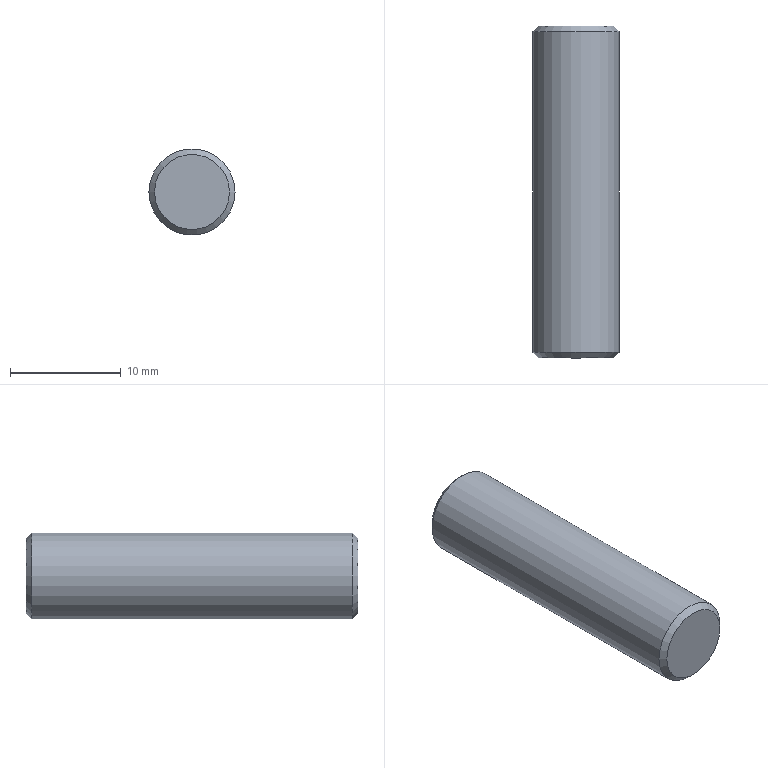Component | NX | STUD_2 | 1 solid | 5 faces | box 7.79 x 30 x 7.79 mm | volume 1422 mm3 | plane 2 | cone 2 | cylinder 1 | commonest cylinder face diameters 7.785 x1
STEP:
#1=CARTESIAN_POINT('',(0.,0.,0.));
#2=DIRECTION('',(0.,0.,1.));
#3=DIRECTION('',(1.,0.,0.));
#4=AXIS2_PLACEMENT_3D('',#1,#2,#3);
#5=CARTESIAN_POINT('',(-23.607,51.5,10.75));
#6=VERTEX_POINT('',#5);
#7=CARTESIAN_POINT('',(-27.,51.5,10.75));
#8=DIRECTION('',(0.,1.,0.));
#9=DIRECTION('',(1.,0.,0.));
#10=AXIS2_PLACEMENT_3D('',#7,#8,#9);
#11=CIRCLE('',#10,3.393);
#12=CARTESIAN_POINT('',(-27.,51.5,10.75));
#13=DIRECTION('',(0.,1.,0.));
#14=DIRECTION('',(1.,0.,0.));
#15=AXIS2_PLACEMENT_3D('',#12,#13,#14);
#16=PLANE('',#15);
#17=CARTESIAN_POINT('',(0.,0.));
#18=DIRECTION('',(1.,0.));
#19=AXIS2_PLACEMENT_2D('',#17,#18);
#20=CIRCLE('',#19,3.393);
#21=(GEOMETRIC_REPRESENTATION_CONTEXT(2)PARAMETRIC_REPRESENTATION_CONTEXT()REPRESENTATION_CONTEXT('',''));
#22=DEFINITIONAL_REPRESENTATION('',(#20),#21);
#23=PCURVE('',#16,#22);
#24=CARTESIAN_POINT('',(-27.,51.,10.75));
#25=DIRECTION('',(0.,-1.,0.));
#26=DIRECTION('',(-1.,0.,0.));
#27=AXIS2_PLACEMENT_3D('',#24,#25,#26);
#28=CONICAL_SURFACE('',#27,3.893,0.7854);
#29=CARTESIAN_POINT('',(9.425,-0.5));
#30=DIRECTION('',(-1.,0.));
#31=VECTOR('',#30,1.);
#32=LINE('',#29,#31);
#33=(GEOMETRIC_REPRESENTATION_CONTEXT(2)PARAMETRIC_REPRESENTATION_CONTEXT()REPRESENTATION_CONTEXT('',''));
#34=DEFINITIONAL_REPRESENTATION('',(#32),#33);
#35=PCURVE('',#28,#34);
#36=SURFACE_CURVE('',#11,(#23,#35),.PCURVE_S1.);
#37=EDGE_CURVE('',#6,#6,#36,.T.);
#38=ORIENTED_EDGE('',*,*,#37,.T.);
#39=EDGE_LOOP('',(#38));
#40=FACE_BOUND('',#39,.T.);
#41=ADVANCED_FACE('',(#40),#16,.T.);
#42=CARTESIAN_POINT('',(-30.393,21.5,10.75));
#43=VERTEX_POINT('',#42);
#44=CARTESIAN_POINT('',(-27.,21.5,10.75));
#45=DIRECTION('',(0.,-1.,0.));
#46=DIRECTION('',(-1.,0.,0.));
#47=AXIS2_PLACEMENT_3D('',#44,#45,#46);
#48=CIRCLE('',#47,3.393);
#49=CARTESIAN_POINT('',(-27.,21.5,10.75));
#50=DIRECTION('',(0.,-1.,0.));
#51=DIRECTION('',(-1.,0.,0.));
#52=AXIS2_PLACEMENT_3D('',#49,#50,#51);
#53=PLANE('',#52);
#54=CARTESIAN_POINT('',(0.,0.));
#55=DIRECTION('',(1.,0.));
#56=AXIS2_PLACEMENT_2D('',#54,#55);
#57=CIRCLE('',#56,3.393);
#58=(GEOMETRIC_REPRESENTATION_CONTEXT(2)PARAMETRIC_REPRESENTATION_CONTEXT()REPRESENTATION_CONTEXT('',''));
#59=DEFINITIONAL_REPRESENTATION('',(#57),#58);
#60=PCURVE('',#53,#59);
#61=CARTESIAN_POINT('',(-27.,22.,10.75));
#62=DIRECTION('',(0.,1.,0.));
#63=DIRECTION('',(1.,0.,0.));
#64=AXIS2_PLACEMENT_3D('',#61,#62,#63);
#65=CONICAL_SURFACE('',#64,3.893,0.7854);
#66=CARTESIAN_POINT('',(9.425,-0.5));
#67=DIRECTION('',(-1.,0.));
#68=VECTOR('',#67,1.);
#69=LINE('',#66,#68);
#70=(GEOMETRIC_REPRESENTATION_CONTEXT(2)PARAMETRIC_REPRESENTATION_CONTEXT()REPRESENTATION_CONTEXT('',''));
#71=DEFINITIONAL_REPRESENTATION('',(#69),#70);
#72=PCURVE('',#65,#71);
#73=SURFACE_CURVE('',#48,(#60,#72),.PCURVE_S1.);
#74=EDGE_CURVE('',#43,#43,#73,.T.);
#75=ORIENTED_EDGE('',*,*,#74,.T.);
#76=EDGE_LOOP('',(#75));
#77=FACE_BOUND('',#76,.T.);
#78=ADVANCED_FACE('',(#77),#53,.T.);
#79=CARTESIAN_POINT('',(-30.893,22.,10.75));
#80=VERTEX_POINT('',#79);
#81=CARTESIAN_POINT('',(-23.107,22.,10.75));
#82=VERTEX_POINT('',#81);
#83=CARTESIAN_POINT('',(-27.,22.,10.75));
#84=DIRECTION('',(0.,1.,0.));
#85=DIRECTION('',(-1.,0.,0.));
#86=AXIS2_PLACEMENT_3D('',#83,#84,#85);
#87=CIRCLE('',#86,3.893);
#88=CARTESIAN_POINT('',(-27.,21.5,10.75));
#89=DIRECTION('',(0.,1.,0.));
#90=DIRECTION('',(1.,0.,0.));
#91=AXIS2_PLACEMENT_3D('',#88,#89,#90);
#92=CYLINDRICAL_SURFACE('',#91,3.893);
#93=CARTESIAN_POINT('',(3.142,0.5));
#94=DIRECTION('',(1.,0.));
#95=VECTOR('',#94,1.);
#96=LINE('',#93,#95);
#97=(GEOMETRIC_REPRESENTATION_CONTEXT(2)PARAMETRIC_REPRESENTATION_CONTEXT()REPRESENTATION_CONTEXT('',''));
#98=DEFINITIONAL_REPRESENTATION('',(#96),#97);
#99=PCURVE('',#92,#98);
#100=CARTESIAN_POINT('',(3.142,0.));
#101=DIRECTION('',(1.,0.));
#102=VECTOR('',#101,1.);
#103=LINE('',#100,#102);
#104=(GEOMETRIC_REPRESENTATION_CONTEXT(2)PARAMETRIC_REPRESENTATION_CONTEXT()REPRESENTATION_CONTEXT('',''));
#105=DEFINITIONAL_REPRESENTATION('',(#103),#104);
#106=PCURVE('',#65,#105);
#107=SURFACE_CURVE('',#87,(#99,#106),.PCURVE_S1.);
#108=EDGE_CURVE('',#80,#82,#107,.T.);
#109=ORIENTED_EDGE('',*,*,#108,.T.);
#110=CARTESIAN_POINT('',(-23.107,51.,10.75));
#111=VERTEX_POINT('',#110);
#112=CARTESIAN_POINT('',(-23.107,22.,10.75));
#113=CARTESIAN_POINT('',(-23.107,51.,10.75));
#114=B_SPLINE_CURVE_WITH_KNOTS('',1,(#112,#113),.UNSPECIFIED.,.F.,.F.,(2,2),(0.5,29.5),.PIECEWISE_BEZIER_KNOTS.);
#115=CARTESIAN_POINT('',(6.283,0.));
#116=DIRECTION('',(0.,1.));
#117=VECTOR('',#116,1.);
#118=LINE('',#115,#117);
#119=(GEOMETRIC_REPRESENTATION_CONTEXT(2)PARAMETRIC_REPRESENTATION_CONTEXT()REPRESENTATION_CONTEXT('',''));
#120=DEFINITIONAL_REPRESENTATION('',(#118),#119);
#121=PCURVE('',#92,#120);
#122=CARTESIAN_POINT('',(0.,0.));
#123=DIRECTION('',(0.,1.));
#124=VECTOR('',#123,1.);
#125=LINE('',#122,#124);
#126=(GEOMETRIC_REPRESENTATION_CONTEXT(2)PARAMETRIC_REPRESENTATION_CONTEXT()REPRESENTATION_CONTEXT('',''));
#127=DEFINITIONAL_REPRESENTATION('',(#125),#126);
#128=PCURVE('',#92,#127);
#129=SEAM_CURVE('',#114,(#121,#128),.PCURVE_S1.);
#130=EDGE_CURVE('',#82,#111,#129,.T.);
#131=ORIENTED_EDGE('',*,*,#130,.T.);
#132=CARTESIAN_POINT('',(-27.,51.,10.75));
#133=DIRECTION('',(0.,-1.,0.));
#134=DIRECTION('',(1.,0.,0.));
#135=AXIS2_PLACEMENT_3D('',#132,#133,#134);
#136=CIRCLE('',#135,3.893);
#137=CARTESIAN_POINT('',(6.283,29.5));
#138=DIRECTION('',(-1.,0.));
#139=VECTOR('',#138,1.);
#140=LINE('',#137,#139);
#141=(GEOMETRIC_REPRESENTATION_CONTEXT(2)PARAMETRIC_REPRESENTATION_CONTEXT()REPRESENTATION_CONTEXT('',''));
#142=DEFINITIONAL_REPRESENTATION('',(#140),#141);
#143=PCURVE('',#92,#142);
#144=CARTESIAN_POINT('',(3.142,0.));
#145=DIRECTION('',(1.,0.));
#146=VECTOR('',#145,1.);
#147=LINE('',#144,#146);
#148=(GEOMETRIC_REPRESENTATION_CONTEXT(2)PARAMETRIC_REPRESENTATION_CONTEXT()REPRESENTATION_CONTEXT('',''));
#149=DEFINITIONAL_REPRESENTATION('',(#147),#148);
#150=PCURVE('',#28,#149);
#151=SURFACE_CURVE('',#136,(#143,#150),.PCURVE_S1.);
#152=EDGE_CURVE('',#111,#111,#151,.T.);
#153=ORIENTED_EDGE('',*,*,#152,.T.);
#154=ORIENTED_EDGE('',*,*,#130,.F.);
#155=CARTESIAN_POINT('',(-27.,22.,10.75));
#156=DIRECTION('',(0.,1.,0.));
#157=DIRECTION('',(-1.,0.,0.));
#158=AXIS2_PLACEMENT_3D('',#155,#156,#157);
#159=CIRCLE('',#158,3.893);
#160=CARTESIAN_POINT('',(-3.142,0.5));
#161=DIRECTION('',(1.,0.));
#162=VECTOR('',#161,1.);
#163=LINE('',#160,#162);
#164=(GEOMETRIC_REPRESENTATION_CONTEXT(2)PARAMETRIC_REPRESENTATION_CONTEXT()REPRESENTATION_CONTEXT('',''));
#165=DEFINITIONAL_REPRESENTATION('',(#163),#164);
#166=PCURVE('',#92,#165);
#167=CARTESIAN_POINT('',(3.142,0.));
#168=DIRECTION('',(1.,0.));
#169=VECTOR('',#168,1.);
#170=LINE('',#167,#169);
#171=(GEOMETRIC_REPRESENTATION_CONTEXT(2)PARAMETRIC_REPRESENTATION_CONTEXT()REPRESENTATION_CONTEXT('',''));
#172=DEFINITIONAL_REPRESENTATION('',(#170),#171);
#173=PCURVE('',#65,#172);
#174=SURFACE_CURVE('',#159,(#166,#173),.PCURVE_S1.);
#175=EDGE_CURVE('',#82,#80,#174,.T.);
#176=ORIENTED_EDGE('',*,*,#175,.T.);
#177=EDGE_LOOP('',(#109,#131,#153,#154,#176));
#178=FACE_BOUND('',#177,.T.);
#179=ADVANCED_FACE('',(#178),#92,.T.);
#180=ORIENTED_EDGE('',*,*,#74,.F.);
#181=CARTESIAN_POINT('',(-30.393,21.5,10.75));
#182=CARTESIAN_POINT('',(-30.893,22.,10.75));
#183=B_SPLINE_CURVE_WITH_KNOTS('',1,(#181,#182),.UNSPECIFIED.,.F.,.F.,(2,2),(-0.7071,0.),.PIECEWISE_BEZIER_KNOTS.);
#184=CARTESIAN_POINT('',(9.425,0.));
#185=DIRECTION('',(0.,1.));
#186=VECTOR('',#185,1.);
#187=LINE('',#184,#186);
#188=(GEOMETRIC_REPRESENTATION_CONTEXT(2)PARAMETRIC_REPRESENTATION_CONTEXT()REPRESENTATION_CONTEXT('',''));
#189=DEFINITIONAL_REPRESENTATION('',(#187),#188);
#190=PCURVE('',#65,#189);
#191=CARTESIAN_POINT('',(3.142,0.));
#192=DIRECTION('',(0.,1.));
#193=VECTOR('',#192,1.);
#194=LINE('',#191,#193);
#195=(GEOMETRIC_REPRESENTATION_CONTEXT(2)PARAMETRIC_REPRESENTATION_CONTEXT()REPRESENTATION_CONTEXT('',''));
#196=DEFINITIONAL_REPRESENTATION('',(#194),#195);
#197=PCURVE('',#65,#196);
#198=SEAM_CURVE('',#183,(#190,#197),.PCURVE_S1.);
#199=EDGE_CURVE('',#43,#80,#198,.T.);
#200=ORIENTED_EDGE('',*,*,#199,.T.);
#201=ORIENTED_EDGE('',*,*,#175,.F.);
#202=ORIENTED_EDGE('',*,*,#108,.F.);
#203=ORIENTED_EDGE('',*,*,#199,.F.);
#204=EDGE_LOOP('',(#180,#200,#201,#202,#203));
#205=FACE_BOUND('',#204,.T.);
#206=ADVANCED_FACE('',(#205),#65,.T.);
#207=ORIENTED_EDGE('',*,*,#37,.F.);
#208=CARTESIAN_POINT('',(-23.607,51.5,10.75));
#209=CARTESIAN_POINT('',(-23.107,51.,10.75));
#210=B_SPLINE_CURVE_WITH_KNOTS('',1,(#208,#209),.UNSPECIFIED.,.F.,.F.,(2,2),(-0.7071,0.),.PIECEWISE_BEZIER_KNOTS.);
#211=CARTESIAN_POINT('',(9.425,0.));
#212=DIRECTION('',(0.,1.));
#213=VECTOR('',#212,1.);
#214=LINE('',#211,#213);
#215=(GEOMETRIC_REPRESENTATION_CONTEXT(2)PARAMETRIC_REPRESENTATION_CONTEXT()REPRESENTATION_CONTEXT('',''));
#216=DEFINITIONAL_REPRESENTATION('',(#214),#215);
#217=PCURVE('',#28,#216);
#218=CARTESIAN_POINT('',(3.142,0.));
#219=DIRECTION('',(0.,1.));
#220=VECTOR('',#219,1.);
#221=LINE('',#218,#220);
#222=(GEOMETRIC_REPRESENTATION_CONTEXT(2)PARAMETRIC_REPRESENTATION_CONTEXT()REPRESENTATION_CONTEXT('',''));
#223=DEFINITIONAL_REPRESENTATION('',(#221),#222);
#224=PCURVE('',#28,#223);
#225=SEAM_CURVE('',#210,(#217,#224),.PCURVE_S1.);
#226=EDGE_CURVE('',#6,#111,#225,.T.);
#227=ORIENTED_EDGE('',*,*,#226,.T.);
#228=ORIENTED_EDGE('',*,*,#152,.F.);
#229=ORIENTED_EDGE('',*,*,#226,.F.);
#230=EDGE_LOOP('',(#207,#227,#228,#229));
#231=FACE_BOUND('',#230,.T.);
#232=ADVANCED_FACE('',(#231),#28,.T.);
#233=CLOSED_SHELL('',(#41,#78,#179,#206,#232));
#234=MANIFOLD_SOLID_BREP('',#233);
#235=(LENGTH_UNIT()NAMED_UNIT(*)SI_UNIT(.MILLI.,.METRE.));
#236=UNCERTAINTY_MEASURE_WITH_UNIT(LENGTH_MEASURE(0.00001),#235,'','');
#237=(NAMED_UNIT(*)PLANE_ANGLE_UNIT()SI_UNIT($,.RADIAN.));
#238=(NAMED_UNIT(*)SI_UNIT($,.STERADIAN.)SOLID_ANGLE_UNIT());
#239=(GEOMETRIC_REPRESENTATION_CONTEXT(3)GLOBAL_UNCERTAINTY_ASSIGNED_CONTEXT((#236))GLOBAL_UNIT_ASSIGNED_CONTEXT((#235,#237,#238))REPRESENTATION_CONTEXT('',''));
#240=ADVANCED_BREP_SHAPE_REPRESENTATION('',(#4,#234),#239);